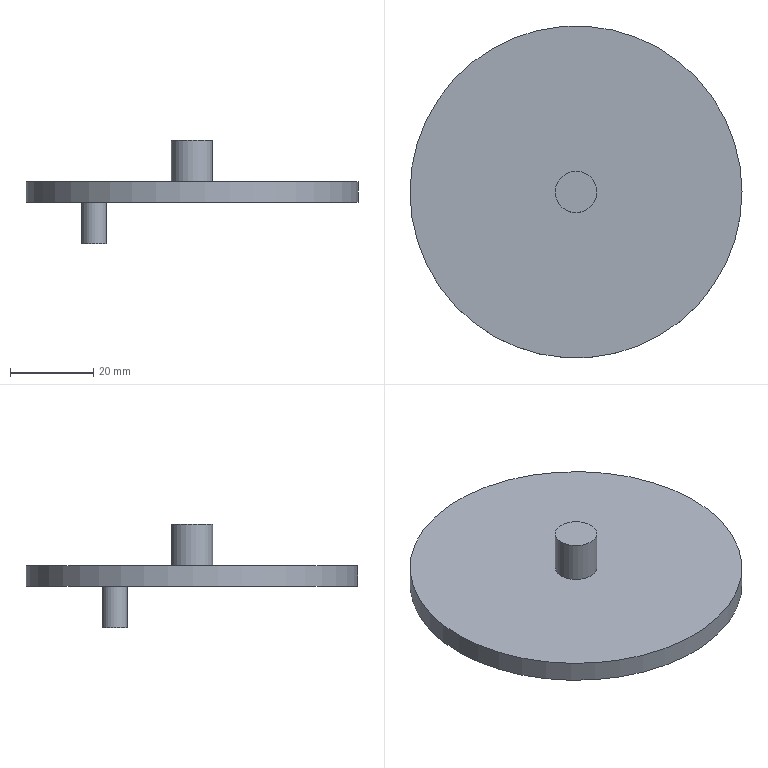Component | NX | ROUND_DISC | 1 solid | 7 faces | box 80 x 80 x 25 mm | volume 26201 mm3 | plane 4 | cylinder 3 | commonest cylinder face diameters 80 x1 10 x1 6 x1
STEP:
#1=CARTESIAN_POINT('',(0.,0.,0.));
#2=DIRECTION('',(0.,0.,1.));
#3=DIRECTION('',(1.,0.,0.));
#4=AXIS2_PLACEMENT_3D('',#1,#2,#3);
#5=CARTESIAN_POINT('',(-24.791,-49.984,7.5));
#6=VERTEX_POINT('',#5);
#7=CARTESIAN_POINT('',(-0.,-18.593,7.5));
#8=DIRECTION('',(0.,0.,1.));
#9=DIRECTION('',(-0.6198,-0.7848,0.));
#10=AXIS2_PLACEMENT_3D('',#7,#8,#9);
#11=CIRCLE('',#10,40.);
#12=CARTESIAN_POINT('',(-0.,-18.593,7.5));
#13=DIRECTION('',(0.,0.,-1.));
#14=DIRECTION('',(0.6198,0.7848,0.));
#15=AXIS2_PLACEMENT_3D('',#12,#13,#14);
#16=CYLINDRICAL_SURFACE('',#15,40.);
#17=CARTESIAN_POINT('',(9.425,0.));
#18=DIRECTION('',(-1.,0.));
#19=VECTOR('',#18,1.);
#20=LINE('',#17,#19);
#21=(GEOMETRIC_REPRESENTATION_CONTEXT(2)PARAMETRIC_REPRESENTATION_CONTEXT()REPRESENTATION_CONTEXT('',''));
#22=DEFINITIONAL_REPRESENTATION('',(#20),#21);
#23=PCURVE('',#16,#22);
#24=CARTESIAN_POINT('',(-0.,-18.593,7.5));
#25=DIRECTION('',(0.,0.,1.));
#26=DIRECTION('',(-0.6198,-0.7848,0.));
#27=AXIS2_PLACEMENT_3D('',#24,#25,#26);
#28=PLANE('',#27);
#29=CARTESIAN_POINT('',(0.,0.));
#30=DIRECTION('',(1.,0.));
#31=AXIS2_PLACEMENT_2D('',#29,#30);
#32=CIRCLE('',#31,40.);
#33=(GEOMETRIC_REPRESENTATION_CONTEXT(2)PARAMETRIC_REPRESENTATION_CONTEXT()REPRESENTATION_CONTEXT('',''));
#34=DEFINITIONAL_REPRESENTATION('',(#32),#33);
#35=PCURVE('',#28,#34);
#36=SURFACE_CURVE('',#11,(#23,#35),.PCURVE_S1.);
#37=EDGE_CURVE('',#6,#6,#36,.T.);
#38=ORIENTED_EDGE('',*,*,#37,.F.);
#39=CARTESIAN_POINT('',(-24.791,-49.984,2.5));
#40=VERTEX_POINT('',#39);
#41=CARTESIAN_POINT('',(-24.791,-49.984,7.5));
#42=CARTESIAN_POINT('',(-24.791,-49.984,2.5));
#43=B_SPLINE_CURVE_WITH_KNOTS('',1,(#41,#42),.UNSPECIFIED.,.F.,.F.,(2,2),(0.,5.),.PIECEWISE_BEZIER_KNOTS.);
#44=CARTESIAN_POINT('',(9.425,0.));
#45=DIRECTION('',(0.,1.));
#46=VECTOR('',#45,1.);
#47=LINE('',#44,#46);
#48=(GEOMETRIC_REPRESENTATION_CONTEXT(2)PARAMETRIC_REPRESENTATION_CONTEXT()REPRESENTATION_CONTEXT('',''));
#49=DEFINITIONAL_REPRESENTATION('',(#47),#48);
#50=PCURVE('',#16,#49);
#51=CARTESIAN_POINT('',(3.142,0.));
#52=DIRECTION('',(0.,1.));
#53=VECTOR('',#52,1.);
#54=LINE('',#51,#53);
#55=(GEOMETRIC_REPRESENTATION_CONTEXT(2)PARAMETRIC_REPRESENTATION_CONTEXT()REPRESENTATION_CONTEXT('',''));
#56=DEFINITIONAL_REPRESENTATION('',(#54),#55);
#57=PCURVE('',#16,#56);
#58=SEAM_CURVE('',#43,(#50,#57),.PCURVE_S1.);
#59=EDGE_CURVE('',#6,#40,#58,.T.);
#60=ORIENTED_EDGE('',*,*,#59,.T.);
#61=CARTESIAN_POINT('',(-0.,-18.593,2.5));
#62=DIRECTION('',(0.,0.,1.));
#63=DIRECTION('',(-0.6198,-0.7848,0.));
#64=AXIS2_PLACEMENT_3D('',#61,#62,#63);
#65=CIRCLE('',#64,40.);
#66=CARTESIAN_POINT('',(9.425,5.));
#67=DIRECTION('',(-1.,0.));
#68=VECTOR('',#67,1.);
#69=LINE('',#66,#68);
#70=(GEOMETRIC_REPRESENTATION_CONTEXT(2)PARAMETRIC_REPRESENTATION_CONTEXT()REPRESENTATION_CONTEXT('',''));
#71=DEFINITIONAL_REPRESENTATION('',(#69),#70);
#72=PCURVE('',#16,#71);
#73=CARTESIAN_POINT('',(-0.,-18.593,2.5));
#74=DIRECTION('',(0.,0.,1.));
#75=DIRECTION('',(-0.6198,-0.7848,0.));
#76=AXIS2_PLACEMENT_3D('',#73,#74,#75);
#77=PLANE('',#76);
#78=CARTESIAN_POINT('',(0.,0.));
#79=DIRECTION('',(1.,0.));
#80=AXIS2_PLACEMENT_2D('',#78,#79);
#81=CIRCLE('',#80,40.);
#82=(GEOMETRIC_REPRESENTATION_CONTEXT(2)PARAMETRIC_REPRESENTATION_CONTEXT()REPRESENTATION_CONTEXT('',''));
#83=DEFINITIONAL_REPRESENTATION('',(#81),#82);
#84=PCURVE('',#77,#83);
#85=SURFACE_CURVE('',#65,(#72,#84),.PCURVE_S1.);
#86=EDGE_CURVE('',#40,#40,#85,.T.);
#87=ORIENTED_EDGE('',*,*,#86,.T.);
#88=ORIENTED_EDGE('',*,*,#59,.F.);
#89=EDGE_LOOP('',(#38,#60,#87,#88));
#90=FACE_BOUND('',#89,.T.);
#91=ADVANCED_FACE('',(#90),#16,.T.);
#92=CARTESIAN_POINT('',(-3.099,-22.517,7.5));
#93=VERTEX_POINT('',#92);
#94=CARTESIAN_POINT('',(-0.,-18.593,7.5));
#95=DIRECTION('',(0.,0.,1.));
#96=DIRECTION('',(-0.6198,-0.7848,0.));
#97=AXIS2_PLACEMENT_3D('',#94,#95,#96);
#98=CIRCLE('',#97,5.);
#99=CARTESIAN_POINT('',(0.,0.));
#100=DIRECTION('',(1.,0.));
#101=AXIS2_PLACEMENT_2D('',#99,#100);
#102=CIRCLE('',#101,5.);
#103=(GEOMETRIC_REPRESENTATION_CONTEXT(2)PARAMETRIC_REPRESENTATION_CONTEXT()REPRESENTATION_CONTEXT('',''));
#104=DEFINITIONAL_REPRESENTATION('',(#102),#103);
#105=PCURVE('',#28,#104);
#106=CARTESIAN_POINT('',(-0.,-18.593,17.5));
#107=DIRECTION('',(0.,0.,-1.));
#108=DIRECTION('',(0.6198,0.7848,0.));
#109=AXIS2_PLACEMENT_3D('',#106,#107,#108);
#110=CYLINDRICAL_SURFACE('',#109,5.);
#111=CARTESIAN_POINT('',(9.425,10.));
#112=DIRECTION('',(-1.,0.));
#113=VECTOR('',#112,1.);
#114=LINE('',#111,#113);
#115=(GEOMETRIC_REPRESENTATION_CONTEXT(2)PARAMETRIC_REPRESENTATION_CONTEXT()REPRESENTATION_CONTEXT('',''));
#116=DEFINITIONAL_REPRESENTATION('',(#114),#115);
#117=PCURVE('',#110,#116);
#118=SURFACE_CURVE('',#98,(#105,#117),.PCURVE_S1.);
#119=EDGE_CURVE('',#93,#93,#118,.T.);
#120=ORIENTED_EDGE('',*,*,#119,.F.);
#121=EDGE_LOOP('',(#120));
#122=FACE_BOUND('',#121,.T.);
#123=ORIENTED_EDGE('',*,*,#37,.T.);
#124=EDGE_LOOP('',(#123));
#125=FACE_BOUND('',#124,.T.);
#126=ADVANCED_FACE('',(#122,#125),#28,.T.);
#127=CARTESIAN_POINT('',(-25.403,-2.354,2.5));
#128=VERTEX_POINT('',#127);
#129=CARTESIAN_POINT('',(-23.543,-0.,2.5));
#130=DIRECTION('',(0.,0.,-1.));
#131=DIRECTION('',(-0.6198,-0.7848,0.));
#132=AXIS2_PLACEMENT_3D('',#129,#130,#131);
#133=CIRCLE('',#132,3.);
#134=CARTESIAN_POINT('',(3.,-30.));
#135=CARTESIAN_POINT('',(3.,-35.196));
#136=CARTESIAN_POINT('',(-1.5,-32.598));
#137=CARTESIAN_POINT('',(-6.,-30.));
#138=CARTESIAN_POINT('',(-1.5,-27.402));
#139=CARTESIAN_POINT('',(3.,-24.804));
#140=CARTESIAN_POINT('',(3.,-30.));
#141=(BOUNDED_CURVE()B_SPLINE_CURVE(2,(#134,#135,#136,#137,#138,#139,#140),.UNSPECIFIED.,.T.,.F.)B_SPLINE_CURVE_WITH_KNOTS((1,2,2,2,2,1),(-2.094,0.,2.094,4.189,6.283,8.378),.UNSPECIFIED.)CURVE()GEOMETRIC_REPRESENTATION_ITEM()RATIONAL_B_SPLINE_CURVE((1.,0.5,1.,0.5,1.,0.5,1.))REPRESENTATION_ITEM(''));
#142=(GEOMETRIC_REPRESENTATION_CONTEXT(2)PARAMETRIC_REPRESENTATION_CONTEXT()REPRESENTATION_CONTEXT('',''));
#143=DEFINITIONAL_REPRESENTATION('',(#141),#142);
#144=PCURVE('',#77,#143);
#145=CARTESIAN_POINT('',(-23.543,-0.,-7.5));
#146=DIRECTION('',(0.,0.,1.));
#147=DIRECTION('',(-0.6198,-0.7848,0.));
#148=AXIS2_PLACEMENT_3D('',#145,#146,#147);
#149=CYLINDRICAL_SURFACE('',#148,3.);
#150=CARTESIAN_POINT('',(6.283,10.));
#151=DIRECTION('',(-1.,0.));
#152=VECTOR('',#151,1.);
#153=LINE('',#150,#152);
#154=(GEOMETRIC_REPRESENTATION_CONTEXT(2)PARAMETRIC_REPRESENTATION_CONTEXT()REPRESENTATION_CONTEXT('',''));
#155=DEFINITIONAL_REPRESENTATION('',(#153),#154);
#156=PCURVE('',#149,#155);
#157=SURFACE_CURVE('',#133,(#144,#156),.PCURVE_S1.);
#158=EDGE_CURVE('',#128,#128,#157,.T.);
#159=ORIENTED_EDGE('',*,*,#158,.F.);
#160=EDGE_LOOP('',(#159));
#161=FACE_BOUND('',#160,.T.);
#162=ORIENTED_EDGE('',*,*,#86,.F.);
#163=EDGE_LOOP('',(#162));
#164=FACE_BOUND('',#163,.T.);
#165=ADVANCED_FACE('',(#161,#164),#77,.F.);
#166=CARTESIAN_POINT('',(-3.099,-22.517,17.5));
#167=VERTEX_POINT('',#166);
#168=CARTESIAN_POINT('',(-0.,-18.593,17.5));
#169=DIRECTION('',(0.,0.,1.));
#170=DIRECTION('',(-0.6198,-0.7848,0.));
#171=AXIS2_PLACEMENT_3D('',#168,#169,#170);
#172=CIRCLE('',#171,5.);
#173=CARTESIAN_POINT('',(9.425,0.));
#174=DIRECTION('',(-1.,0.));
#175=VECTOR('',#174,1.);
#176=LINE('',#173,#175);
#177=(GEOMETRIC_REPRESENTATION_CONTEXT(2)PARAMETRIC_REPRESENTATION_CONTEXT()REPRESENTATION_CONTEXT('',''));
#178=DEFINITIONAL_REPRESENTATION('',(#176),#177);
#179=PCURVE('',#110,#178);
#180=CARTESIAN_POINT('',(-0.,-18.593,17.5));
#181=DIRECTION('',(0.,0.,1.));
#182=DIRECTION('',(-0.6198,-0.7848,0.));
#183=AXIS2_PLACEMENT_3D('',#180,#181,#182);
#184=PLANE('',#183);
#185=CARTESIAN_POINT('',(0.,0.));
#186=DIRECTION('',(1.,0.));
#187=AXIS2_PLACEMENT_2D('',#185,#186);
#188=CIRCLE('',#187,5.);
#189=(GEOMETRIC_REPRESENTATION_CONTEXT(2)PARAMETRIC_REPRESENTATION_CONTEXT()REPRESENTATION_CONTEXT('',''));
#190=DEFINITIONAL_REPRESENTATION('',(#188),#189);
#191=PCURVE('',#184,#190);
#192=SURFACE_CURVE('',#172,(#179,#191),.PCURVE_S1.);
#193=EDGE_CURVE('',#167,#167,#192,.T.);
#194=ORIENTED_EDGE('',*,*,#193,.F.);
#195=CARTESIAN_POINT('',(-3.099,-22.517,17.5));
#196=CARTESIAN_POINT('',(-3.099,-22.517,7.5));
#197=B_SPLINE_CURVE_WITH_KNOTS('',1,(#195,#196),.UNSPECIFIED.,.F.,.F.,(2,2),(0.,10.),.PIECEWISE_BEZIER_KNOTS.);
#198=CARTESIAN_POINT('',(9.425,0.));
#199=DIRECTION('',(0.,1.));
#200=VECTOR('',#199,1.);
#201=LINE('',#198,#200);
#202=(GEOMETRIC_REPRESENTATION_CONTEXT(2)PARAMETRIC_REPRESENTATION_CONTEXT()REPRESENTATION_CONTEXT('',''));
#203=DEFINITIONAL_REPRESENTATION('',(#201),#202);
#204=PCURVE('',#110,#203);
#205=CARTESIAN_POINT('',(3.142,0.));
#206=DIRECTION('',(0.,1.));
#207=VECTOR('',#206,1.);
#208=LINE('',#205,#207);
#209=(GEOMETRIC_REPRESENTATION_CONTEXT(2)PARAMETRIC_REPRESENTATION_CONTEXT()REPRESENTATION_CONTEXT('',''));
#210=DEFINITIONAL_REPRESENTATION('',(#208),#209);
#211=PCURVE('',#110,#210);
#212=SEAM_CURVE('',#197,(#204,#211),.PCURVE_S1.);
#213=EDGE_CURVE('',#167,#93,#212,.T.);
#214=ORIENTED_EDGE('',*,*,#213,.T.);
#215=ORIENTED_EDGE('',*,*,#119,.T.);
#216=ORIENTED_EDGE('',*,*,#213,.F.);
#217=EDGE_LOOP('',(#194,#214,#215,#216));
#218=FACE_BOUND('',#217,.T.);
#219=ADVANCED_FACE('',(#218),#110,.T.);
#220=ORIENTED_EDGE('',*,*,#193,.T.);
#221=EDGE_LOOP('',(#220));
#222=FACE_BOUND('',#221,.T.);
#223=ADVANCED_FACE('',(#222),#184,.T.);
#224=CARTESIAN_POINT('',(-25.403,-2.354,-7.5));
#225=VERTEX_POINT('',#224);
#226=CARTESIAN_POINT('',(-23.543,-0.,-7.5));
#227=DIRECTION('',(0.,0.,-1.));
#228=DIRECTION('',(-0.6198,-0.7848,0.));
#229=AXIS2_PLACEMENT_3D('',#226,#227,#228);
#230=CIRCLE('',#229,3.);
#231=CARTESIAN_POINT('',(6.283,0.));
#232=DIRECTION('',(-1.,0.));
#233=VECTOR('',#232,1.);
#234=LINE('',#231,#233);
#235=(GEOMETRIC_REPRESENTATION_CONTEXT(2)PARAMETRIC_REPRESENTATION_CONTEXT()REPRESENTATION_CONTEXT('',''));
#236=DEFINITIONAL_REPRESENTATION('',(#234),#235);
#237=PCURVE('',#149,#236);
#238=CARTESIAN_POINT('',(-23.543,-0.,-7.5));
#239=DIRECTION('',(0.,0.,-1.));
#240=DIRECTION('',(0.6198,0.7848,0.));
#241=AXIS2_PLACEMENT_3D('',#238,#239,#240);
#242=PLANE('',#241);
#243=CARTESIAN_POINT('',(0.,0.));
#244=DIRECTION('',(-1.,0.));
#245=AXIS2_PLACEMENT_2D('',#243,#244);
#246=CIRCLE('',#245,3.);
#247=(GEOMETRIC_REPRESENTATION_CONTEXT(2)PARAMETRIC_REPRESENTATION_CONTEXT()REPRESENTATION_CONTEXT('',''));
#248=DEFINITIONAL_REPRESENTATION('',(#246),#247);
#249=PCURVE('',#242,#248);
#250=SURFACE_CURVE('',#230,(#237,#249),.PCURVE_S1.);
#251=EDGE_CURVE('',#225,#225,#250,.T.);
#252=ORIENTED_EDGE('',*,*,#251,.F.);
#253=CARTESIAN_POINT('',(-25.403,-2.354,-7.5));
#254=CARTESIAN_POINT('',(-25.403,-2.354,2.5));
#255=B_SPLINE_CURVE_WITH_KNOTS('',1,(#253,#254),.UNSPECIFIED.,.F.,.F.,(2,2),(0.,10.),.PIECEWISE_BEZIER_KNOTS.);
#256=CARTESIAN_POINT('',(6.283,0.));
#257=DIRECTION('',(0.,1.));
#258=VECTOR('',#257,1.);
#259=LINE('',#256,#258);
#260=(GEOMETRIC_REPRESENTATION_CONTEXT(2)PARAMETRIC_REPRESENTATION_CONTEXT()REPRESENTATION_CONTEXT('',''));
#261=DEFINITIONAL_REPRESENTATION('',(#259),#260);
#262=PCURVE('',#149,#261);
#263=CARTESIAN_POINT('',(0.,0.));
#264=DIRECTION('',(0.,1.));
#265=VECTOR('',#264,1.);
#266=LINE('',#263,#265);
#267=(GEOMETRIC_REPRESENTATION_CONTEXT(2)PARAMETRIC_REPRESENTATION_CONTEXT()REPRESENTATION_CONTEXT('',''));
#268=DEFINITIONAL_REPRESENTATION('',(#266),#267);
#269=PCURVE('',#149,#268);
#270=SEAM_CURVE('',#255,(#262,#269),.PCURVE_S1.);
#271=EDGE_CURVE('',#225,#128,#270,.T.);
#272=ORIENTED_EDGE('',*,*,#271,.T.);
#273=ORIENTED_EDGE('',*,*,#158,.T.);
#274=ORIENTED_EDGE('',*,*,#271,.F.);
#275=EDGE_LOOP('',(#252,#272,#273,#274));
#276=FACE_BOUND('',#275,.T.);
#277=ADVANCED_FACE('',(#276),#149,.T.);
#278=ORIENTED_EDGE('',*,*,#251,.T.);
#279=EDGE_LOOP('',(#278));
#280=FACE_BOUND('',#279,.T.);
#281=ADVANCED_FACE('',(#280),#242,.T.);
#282=CLOSED_SHELL('',(#91,#126,#165,#219,#223,#277,#281));
#283=MANIFOLD_SOLID_BREP('',#282);
#284=(LENGTH_UNIT()NAMED_UNIT(*)SI_UNIT(.MILLI.,.METRE.));
#285=UNCERTAINTY_MEASURE_WITH_UNIT(LENGTH_MEASURE(0.00001),#284,'','');
#286=(NAMED_UNIT(*)PLANE_ANGLE_UNIT()SI_UNIT($,.RADIAN.));
#287=(NAMED_UNIT(*)SI_UNIT($,.STERADIAN.)SOLID_ANGLE_UNIT());
#288=(GEOMETRIC_REPRESENTATION_CONTEXT(3)GLOBAL_UNCERTAINTY_ASSIGNED_CONTEXT((#285))GLOBAL_UNIT_ASSIGNED_CONTEXT((#284,#286,#287))REPRESENTATION_CONTEXT('',''));
#289=ADVANCED_BREP_SHAPE_REPRESENTATION('',(#4,#283),#288);